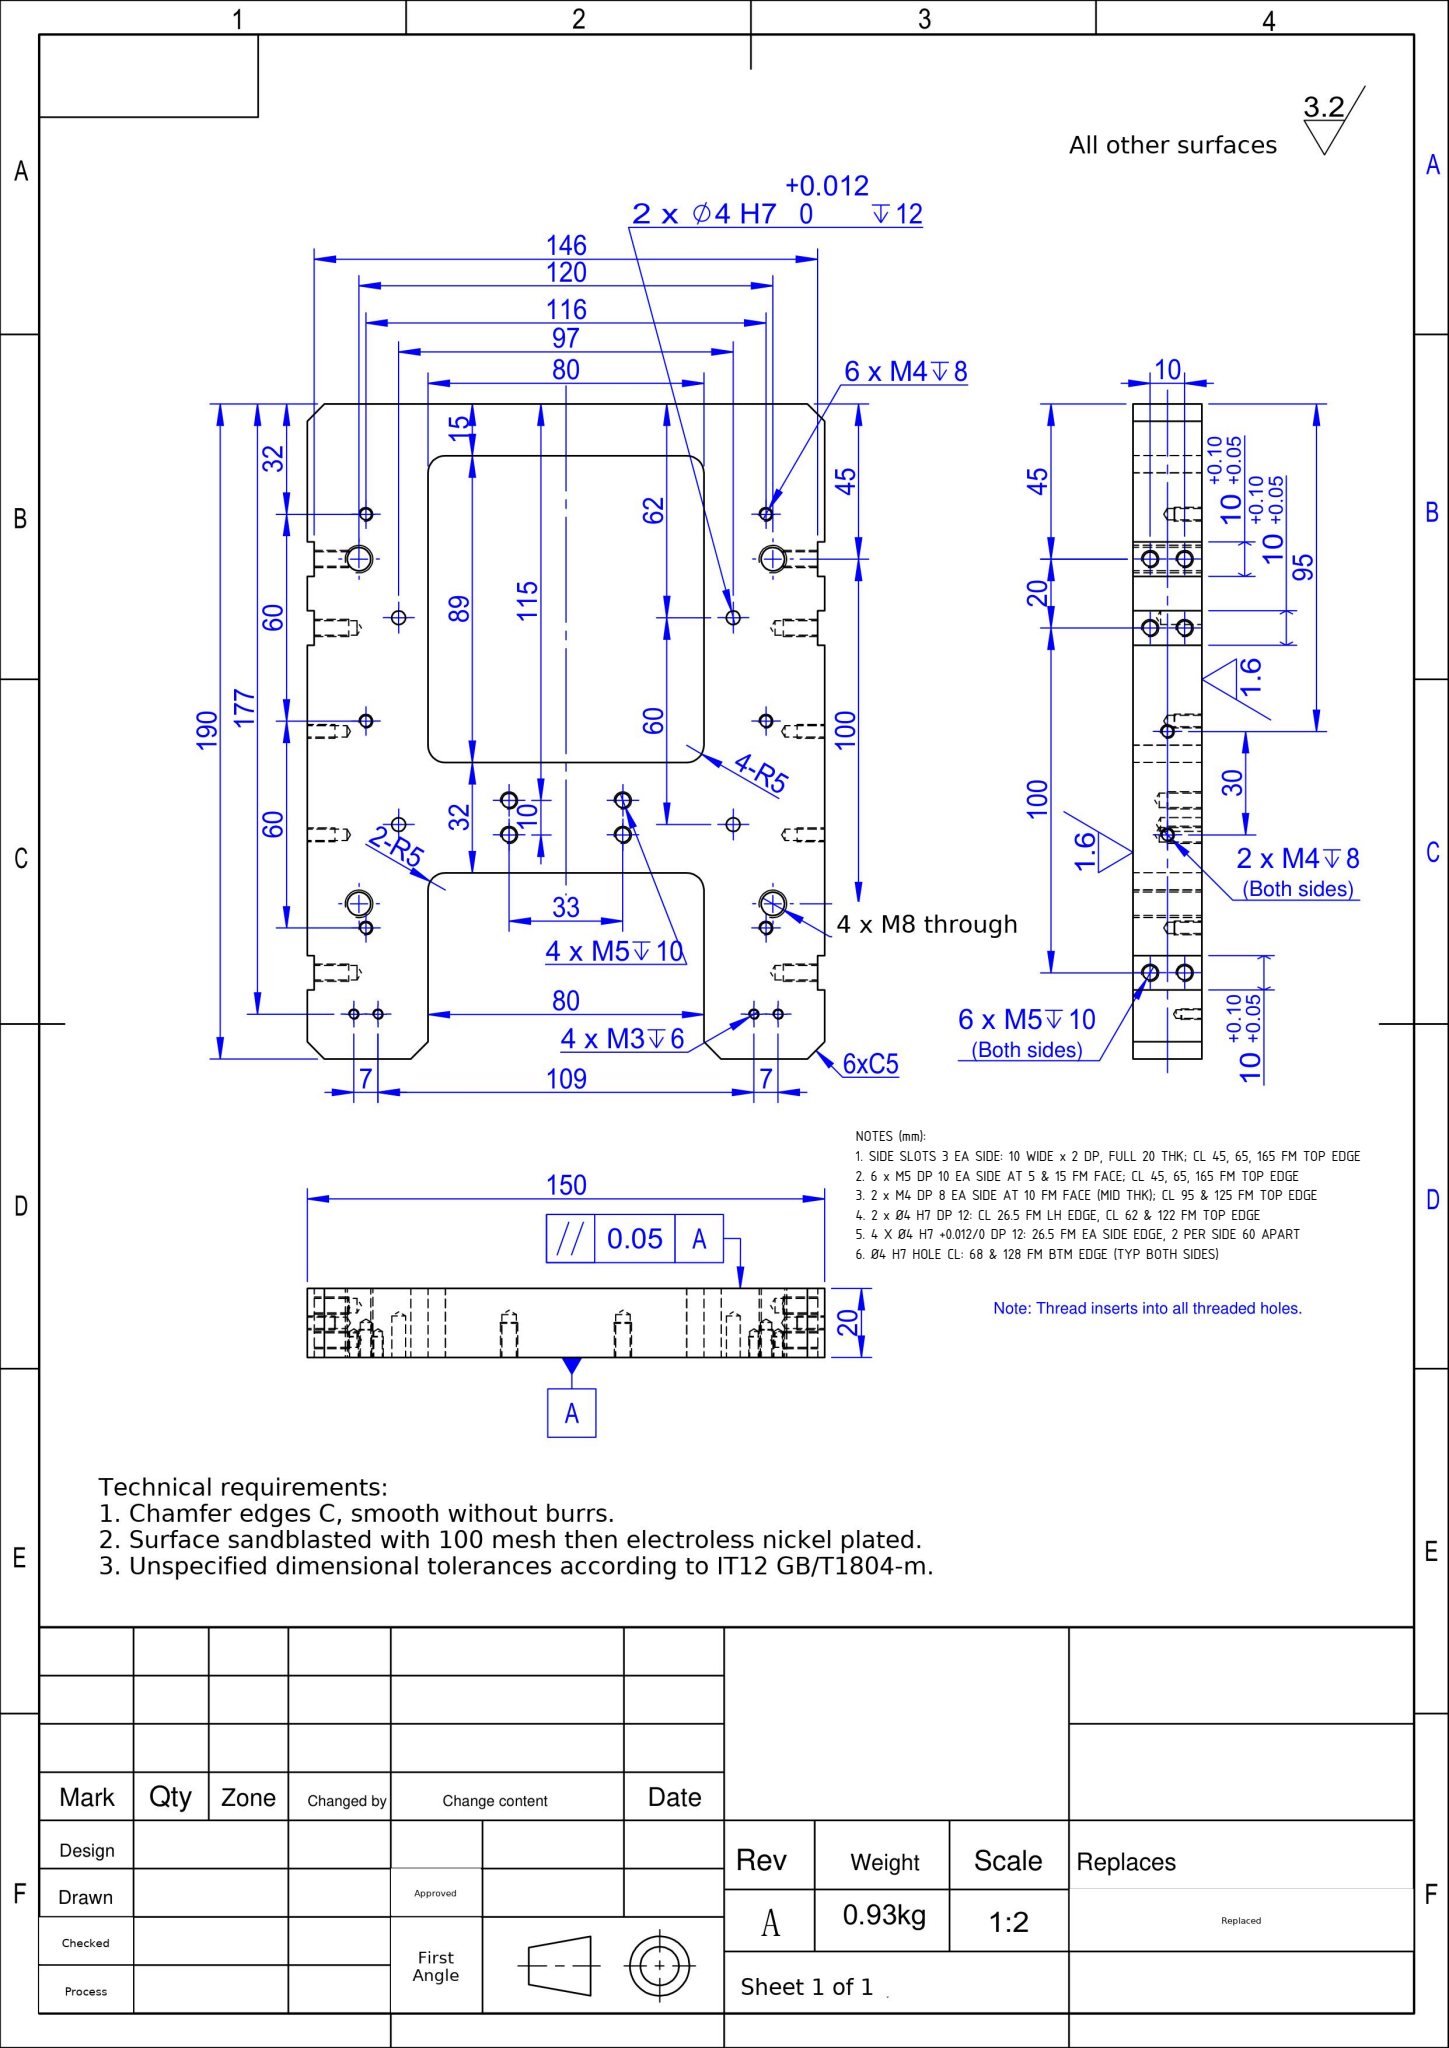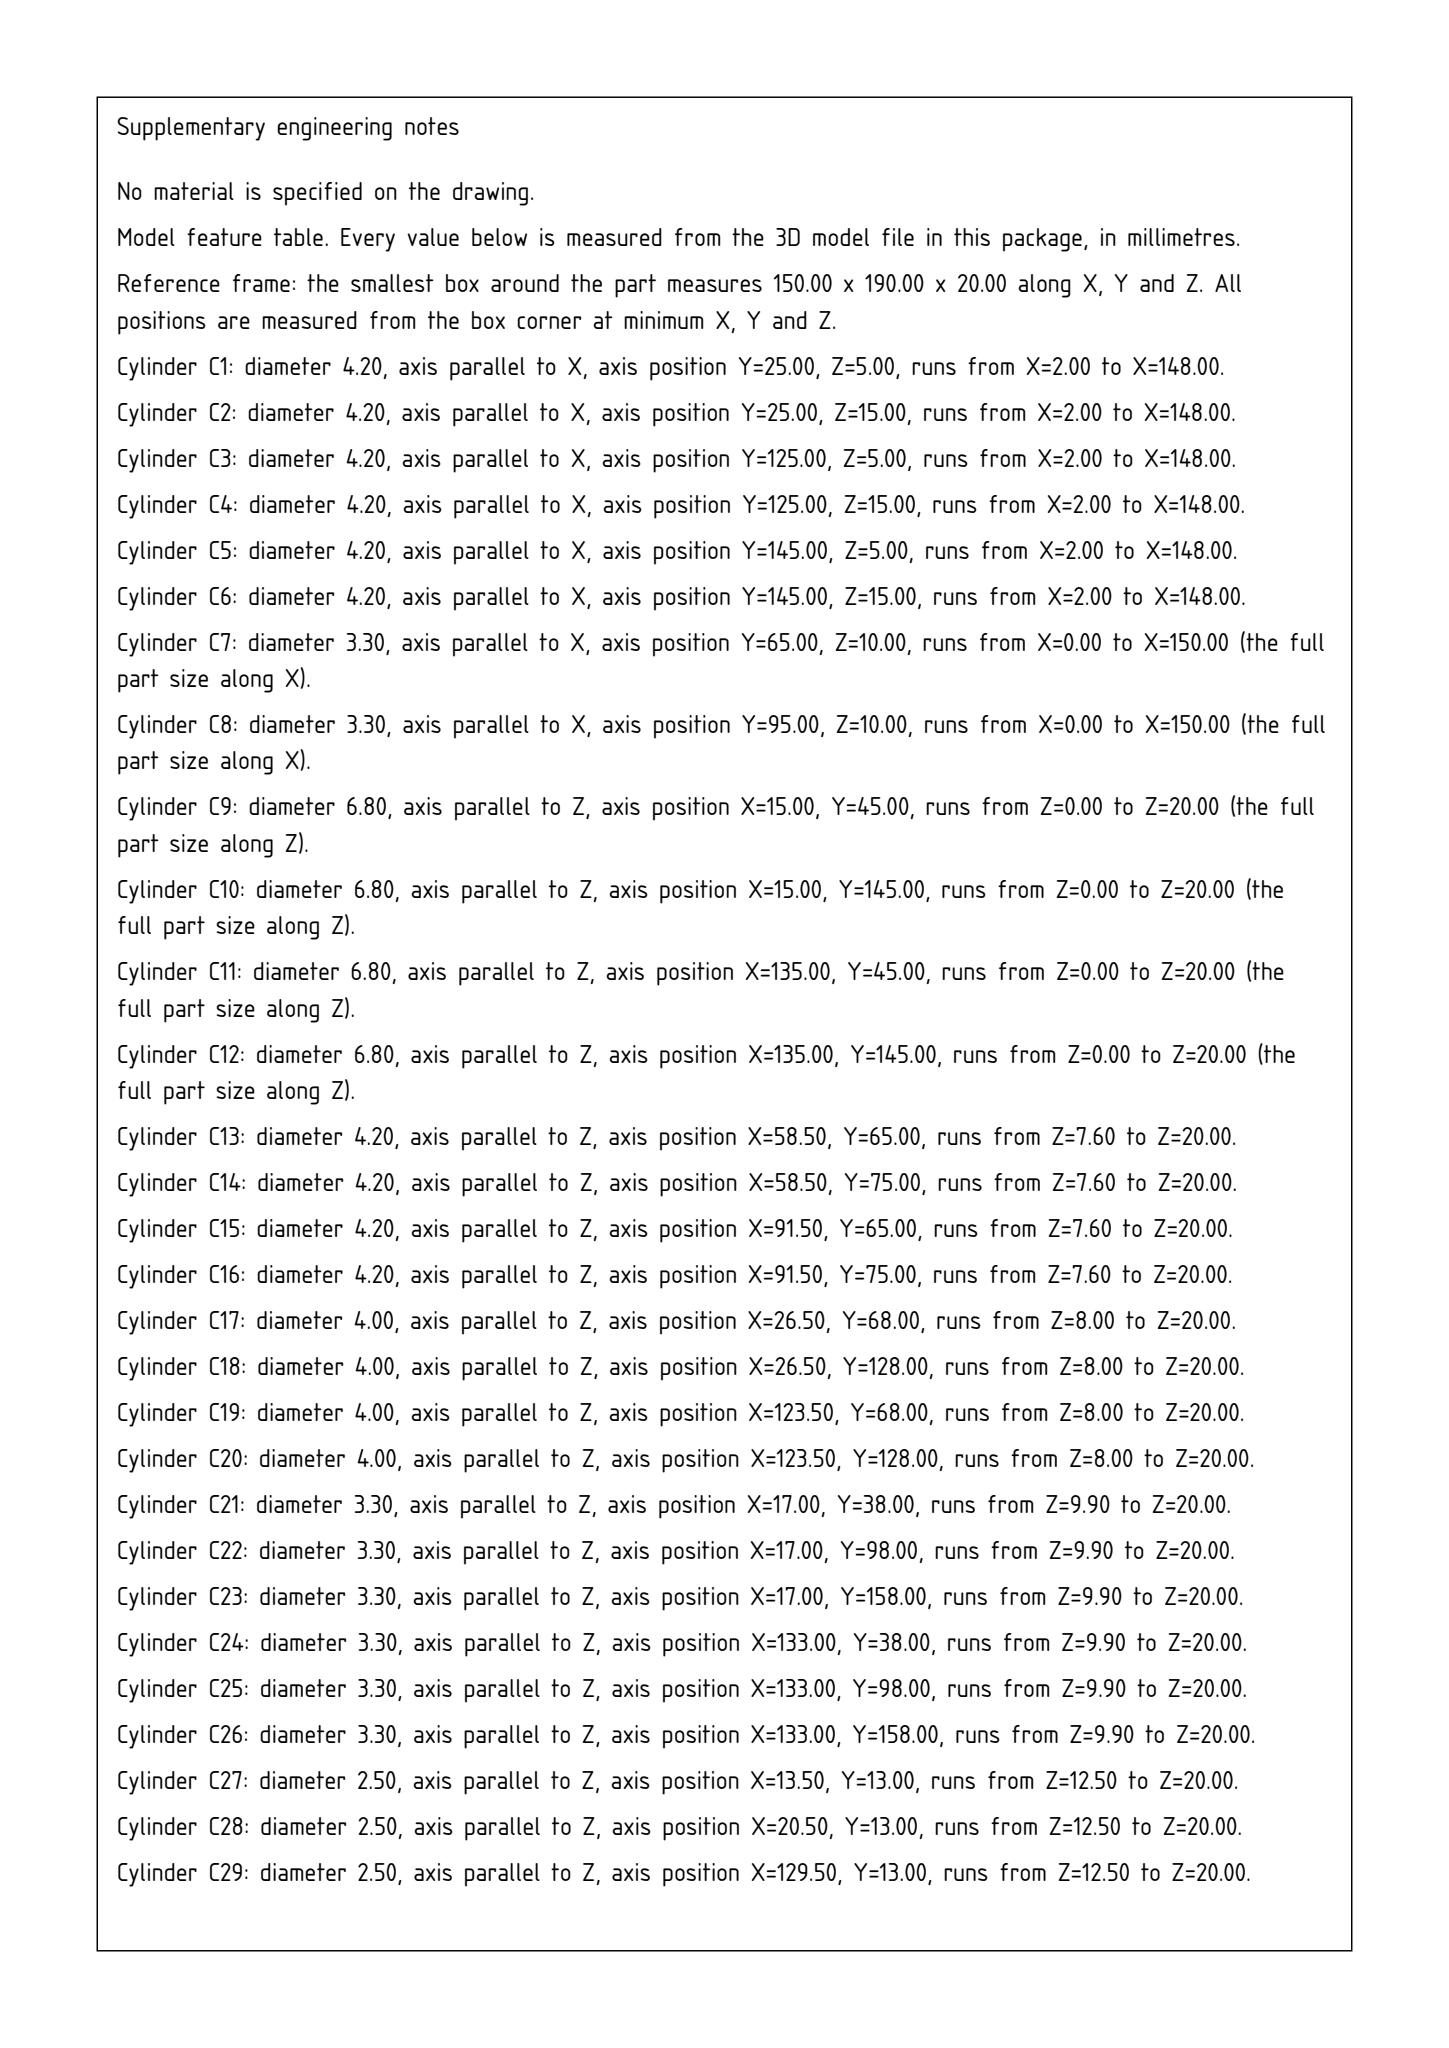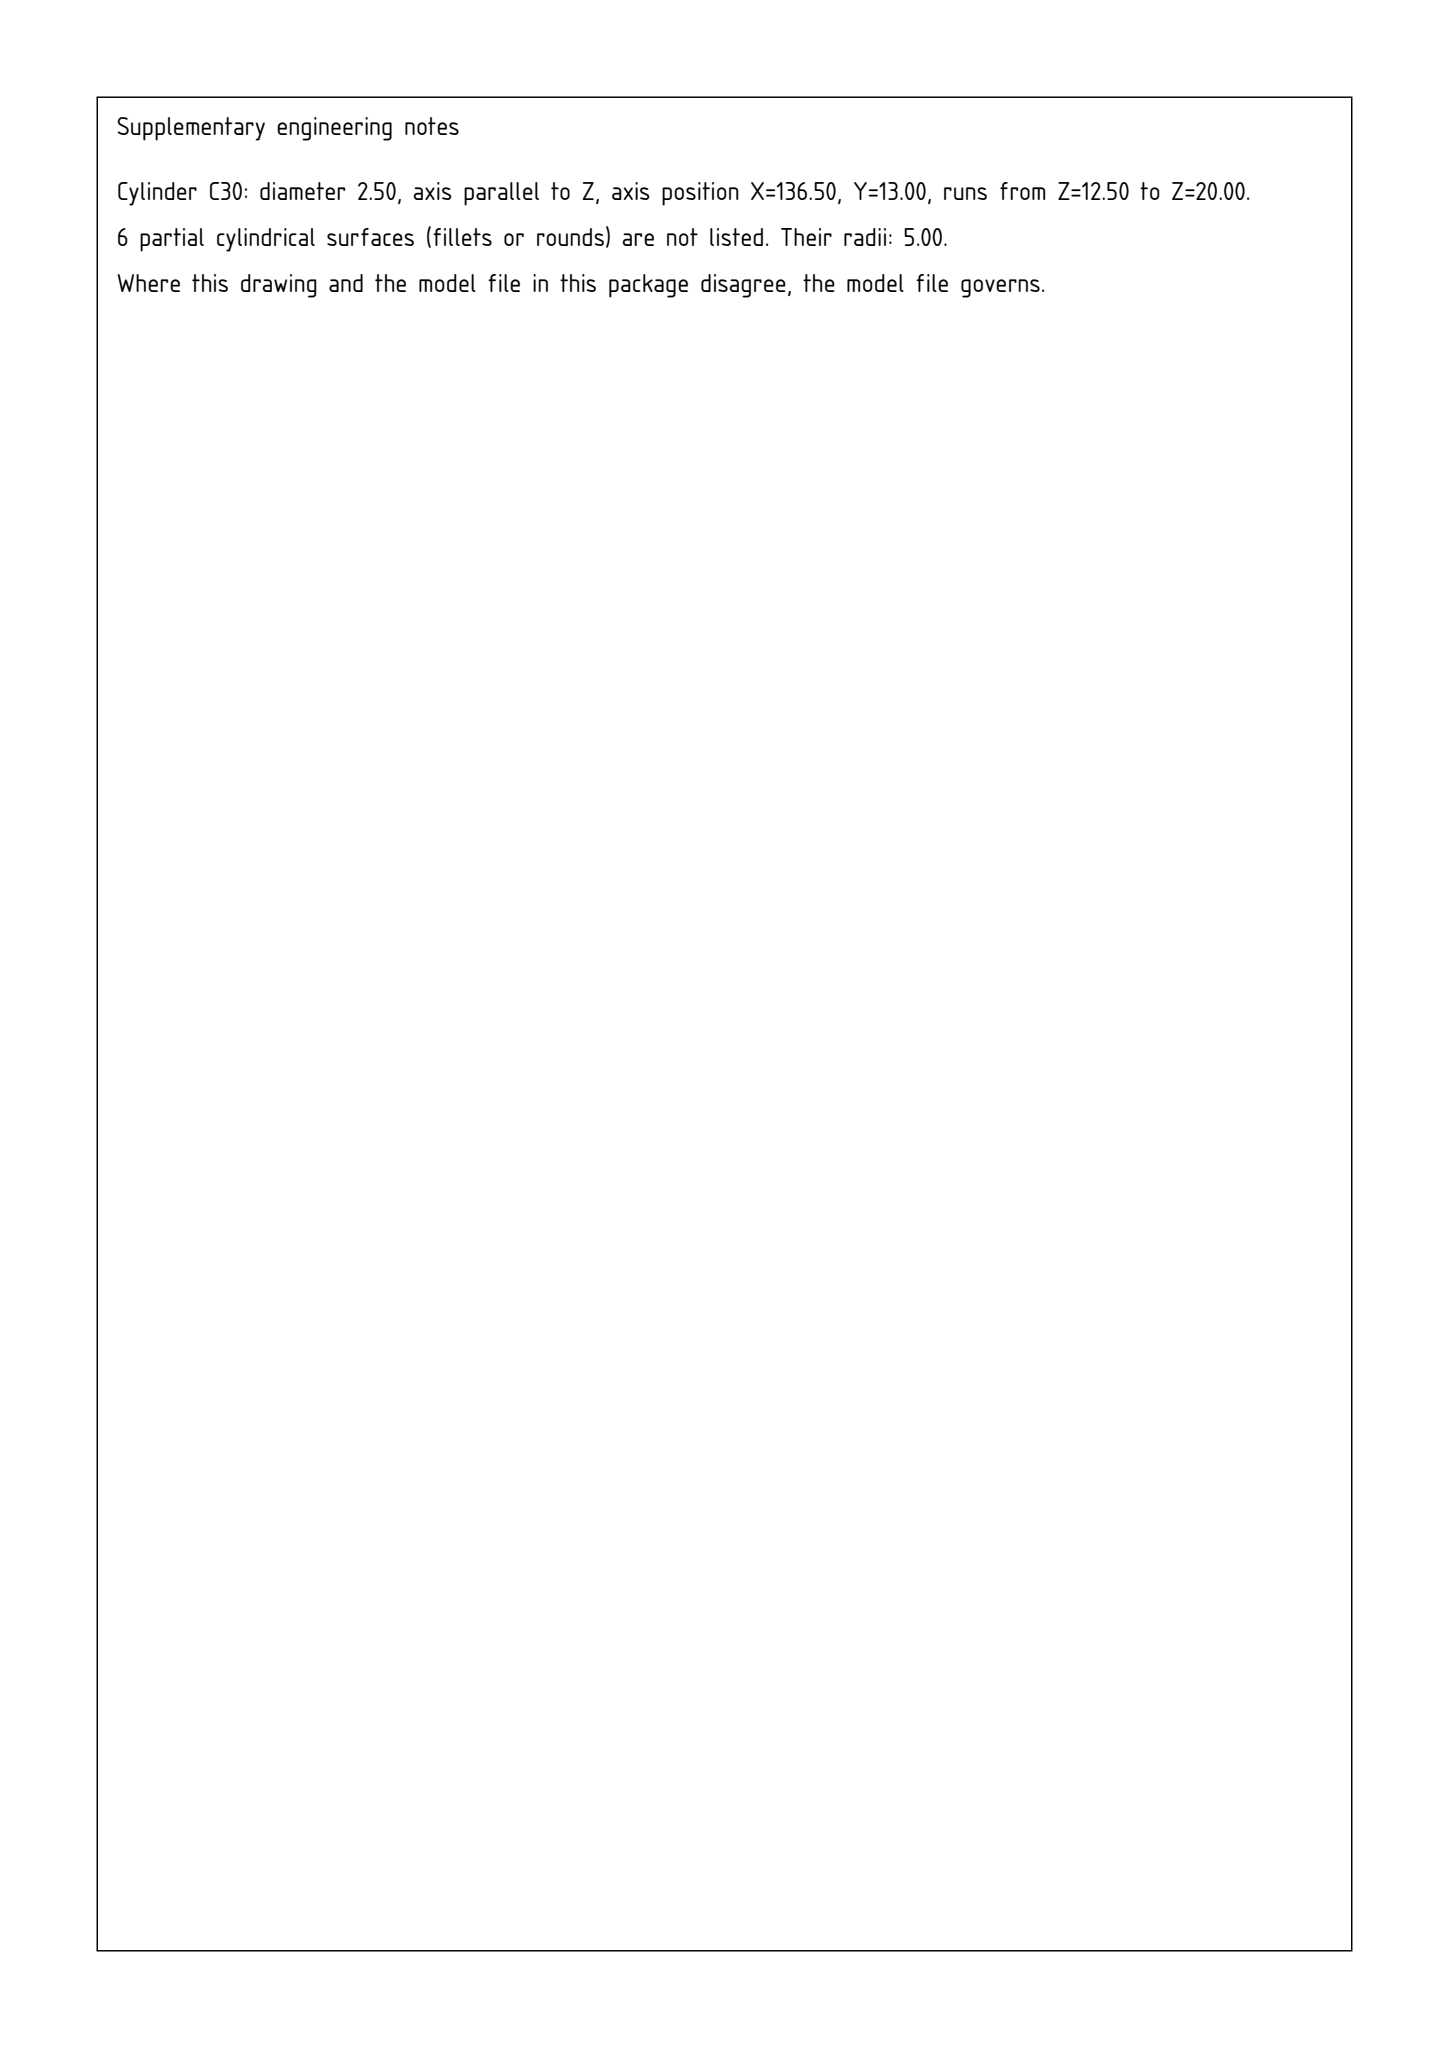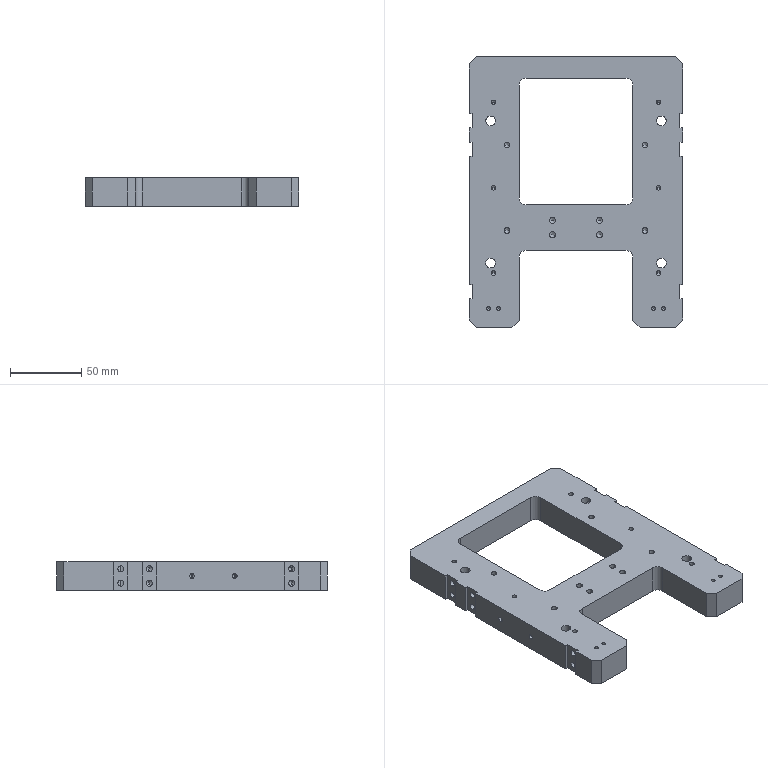Part | SolidWorks | mm | 1 solid | 186 faces | box 150 x 190 x 20 mm | volume 330650 mm3 | cylinder 82 | cone 60 | plane 44 | commonest cylinder face diameters 4.2 x32 3.3 x20 4 x8 6.8 x8 2.5 x8 10 x6
Drawing notes:
SIDE SLOTS 3 EA SIDE: 10 WIDE x 2 DP, FULL 20 THK; CL 45, 65, 165 FM TOP EDGE | from the solid: x-normal planes at 2.0 & 148.0 vs faces x=0/150 -> 2 deep; y pairs 20-30, 120-130, 140-150 -> 10 wide; z 0-20 full thk; slot CL y=145/125/25 -> 190-y = 45/65/165
6 x M5 DP 10 EA SIDE AT 5 & 15 FM FACE; CL 45, 65, 165 FM TOP EDGE | from the solid: Ø4.2 x-axis holes at z=5 and z=15 in 20 thk; at y=145, 125, 25 -> 190-y = 45, 65, 165
2 x M4 DP 8 EA SIDE AT 10 FM FACE (MID THK); CL 95 & 125 FM TOP EDGE | from the solid: Ø3.3 x-axis holes at z=10.0, y=95 and y=65 -> 190-y = 95 and 125
2 x Ø4 H7 DP 12: CL 26.5 FM LH EDGE, CL 62 & 122 FM TOP EDGE | from the solid: dia 4.0 z-holes, x=26.5, y=128 (190-128=62) and y=68 (190-68=122), length 12
4 X Ø4 H7 +0.012/0 DP 12: 26.5 FM EA SIDE EDGE, 2 PER SIDE 60 APART | from the solid: Ø4.0 z-axis holes at (26.5,68),(26.5,128),(123.5,68),(123.5,128), L=12; bbox X=150 so 150-123.5=26.5
Ø4 H7 HOLE CL: 68 & 128 FM BTM EDGE (TYP BOTH SIDES) | from the solid: Ø4.0 holes y=68 and y=128 from bbox Y min; bbox Y=190
build123d program:
from build123d import *

# Parameters (mm, degrees)
SKETCH1_W                         = 150
SKETCH1_H                         = 20
BOSS_EXTRUDE1_DEPTH               = 190
M4_TAPPED_HOLE1_D                 = 3.3
M4_TAPPED_HOLE1_DEPTH             = 10.1
M4_TAPPED_HOLE1_TIP               = 0.9914
M3_TAPPED_HOLE1_D                 = 2.5
M3_TAPPED_HOLE1_DEPTH             = 7.5
M3_TAPPED_HOLE1_TIP               = 0.7511
M5_TAPPED_HOLE1_AT_2_COUNT        = 2
M5_TAPPED_HOLE1_AT_2_PITCH        = 33
CUT_EXTRUDE2_DEPTH                = 206.244
M8_TAPPED_HOLE1_D                 = 6.8
LPATTERN1_COUNT                   = 2
LPATTERN1_PITCH                   = 100
LPATTERN1_COPY_1_D                = 6.8
CHAMFER2_SIZE                     = 5
SKETCH23_W                        = 2
SKETCH23_H                        = 10
CUT_EXTRUDE3_DEPTH                = 206.244
SKETCH24_W                        = 20
SKETCH24_H                        = 10
CUT_EXTRUDE4_DEPTH                = 2
M5_TAPPED_HOLE2_AT_2_COUNT        = 2
M5_TAPPED_HOLE2_AT_2_PITCH        = 10
M5_TAPPED_HOLE2_AT_3_COUNT        = 2
M5_TAPPED_HOLE2_AT_3_PITCH        = 120.416
M5_TAPPED_HOLE2_AT_4_COUNT        = 2
M5_TAPPED_HOLE2_AT_4_PITCH        = 120
M5_TAPPED_HOLE2_AT_5_COUNT        = 2
M5_TAPPED_HOLE2_AT_5_PITCH        = 22.361
M5_TAPPED_HOLE2_AT_6_COUNT        = 2
M5_TAPPED_HOLE2_AT_6_PITCH        = 20
M4_TAPPED_HOLE2_AT_2_COUNT        = 2
M4_TAPPED_HOLE2_AT_2_PITCH        = 30
LPATTERN2_COUNT                   = 2
LPATTERN2_PITCH                   = 10
F_4_0_4_DIAMETER_HOLE1_AT_2_COUNT = 2
F_4_0_4_DIAMETER_HOLE1_AT_2_PITCH = 60


with BuildPart() as part:
    # Sketch1 → Boss-Extrude1 (new body)
    with BuildSketch(Plane(origin=(0, 0, 0), x_dir=(1, 0, 0), z_dir=(0, 1, 0))):
        Rectangle(SKETCH1_W, SKETCH1_H)
    extrude(amount=BOSS_EXTRUDE1_DEPTH)

    # M4 Tapped Hole1
    with Locations(Plane.XY.offset(10)):
        with Locations((-58, 38), (-58, 98), (-58, 158), (58, 158), (58, 98), (58, 38)):
            Hole(M4_TAPPED_HOLE1_D / 2, depth=M4_TAPPED_HOLE1_DEPTH)
            with Locations((0, 0, -(M4_TAPPED_HOLE1_DEPTH + M4_TAPPED_HOLE1_TIP / 2))):  # 118° drill point
                Cone(0, M4_TAPPED_HOLE1_D / 2, M4_TAPPED_HOLE1_TIP, mode=Mode.SUBTRACT)

    # M3 Tapped Hole1
    with Locations(Plane.XY.offset(10)):
        with Locations((54.5, 13), (61.5, 13), (-61.5, 13), (-54.5, 13)):
            Hole(M3_TAPPED_HOLE1_D / 2, depth=M3_TAPPED_HOLE1_DEPTH)
            with Locations((0, 0, -(M3_TAPPED_HOLE1_DEPTH + M3_TAPPED_HOLE1_TIP / 2))):  # 118° drill point
                Cone(0, M3_TAPPED_HOLE1_D / 2, M3_TAPPED_HOLE1_TIP, mode=Mode.SUBTRACT)

    # Sketch9 → M5 Tapped Hole1 (revolve, cut)
    with BuildSketch(Plane(origin=(-16.5, 65, 10), x_dir=(0, -1, 0), z_dir=(1, 0, 0))):
        Polygon((0, 0), (0, 13.662), (2.1, 12.4), (2.1, 0), align=None)
    m5_tapped_hole1 = revolve(axis=Axis((-16.5, 65, 16.35), (0, 0, -1)), mode=Mode.SUBTRACT)

    # M5 Tapped Hole1 at 2: M5 Tapped Hole1 ×2
    with Locations(*[(i * M5_TAPPED_HOLE1_AT_2_PITCH, 0, 0) for i in range(1, M5_TAPPED_HOLE1_AT_2_COUNT)]):
        add(m5_tapped_hole1, mode=Mode.SUBTRACT)

    # Sketch11 → Cut-Extrude2 (cut, through all)
    with BuildSketch(Plane.XY.offset(10)):
        with BuildLine():
            Line((-35, 175), (35, 175))
            ThreePointArc((35, 175), (38.536, 173.536), (40, 170))
            Line((40, 170), (40, 91))
            ThreePointArc((40, 91), (38.536, 87.464), (35, 86))
            Line((35, 86), (-35, 86))
            ThreePointArc((-35, 86), (-38.536, 87.464), (-40, 91))
            Line((-40, 91), (-40, 170))
            ThreePointArc((-40, 170), (-38.536, 173.536), (-35, 175))
        make_face()
        with BuildLine():
            Line((-35, 54), (35, 54))
            ThreePointArc((35, 54), (38.536, 52.536), (40, 49))
            Line((40, 49), (40, 0))
            Line((40, 0), (-40, 0))
            Line((-40, 0), (-40, 49))
            ThreePointArc((-40, 49), (-38.536, 52.536), (-35, 54))
        make_face()
    extrude(amount=-CUT_EXTRUDE2_DEPTH, mode=Mode.SUBTRACT)

    # M8 Tapped Hole1 (through all)
    with Locations(Plane(origin=(116.284, -1.864, 10), x_dir=(-1, 0, 0), z_dir=(0, 0, 1))):
        with Locations((176.284, -146.864)):
            m8_tapped_hole1 = Hole(M8_TAPPED_HOLE1_D / 2)

    # Mirror2: M8 Tapped Hole1 across plane
    add(m8_tapped_hole1.mirror(Plane(origin=(0, 0, 0), x_dir=(0, 0, 1), z_dir=(1, 0, 0))), mode=Mode.SUBTRACT)

    # LPattern1: M8 Tapped Hole1 ×2
    with Locations(*[(0, -i * LPATTERN1_PITCH, 0) for i in range(1, LPATTERN1_COUNT)]):
        add(m8_tapped_hole1, mode=Mode.SUBTRACT)

    # LPattern1 copy 1 (through all)
    with Locations(Plane(origin=(-116.284, -101.864, 10), x_dir=(1, 0, 0), z_dir=(0, 0, 1))):
        with Locations((176.284, 146.864)):
            Hole(LPATTERN1_COPY_1_D / 2)

    # Chamfer2
    chamfer2_edges = [part.edges().sort_by_distance(p)[0] for p in [
        (75, 190, 0),
        (-75, 190, 0),
        (75, 0, 0),
        (-75, 0, 0),
        (40, 0, 0),
        (-40, 0, 0),
    ]]
    chamfer(chamfer2_edges, length=CHAMFER2_SIZE)

    # Sketch23 → Cut-Extrude3 (cut, through all)
    with BuildSketch(Plane.XY.offset(10)):
        with Locations((-74, 25)):
            Rectangle(SKETCH23_W, SKETCH23_H)
    cut_extrude3 = extrude(amount=-CUT_EXTRUDE3_DEPTH, mode=Mode.SUBTRACT)

    # Sketch24 → Cut-Extrude4 (cut)
    with BuildSketch(Plane.ZY.offset(75)):
        with Locations((0, 145)):
            Rectangle(SKETCH24_W, SKETCH24_H)
        with Locations((0, 125)):
            Rectangle(SKETCH24_W, SKETCH24_H)
    cut_extrude4 = extrude(amount=-CUT_EXTRUDE4_DEPTH, mode=Mode.SUBTRACT)

    # Sketch25 → M5 Tapped Hole2 (revolve, cut)
    with BuildSketch(Plane(origin=(-73, 145, 5), x_dir=(0, 0, 1), z_dir=(0, 1, 0))):
        Polygon((0, 0), (0, 13.662), (2.1, 12.4), (2.1, 0), align=None)
    m5_tapped_hole2 = revolve(axis=Axis((-79.35, 145, 5), (1, 0, 0)), mode=Mode.SUBTRACT)

    # M5 Tapped Hole2 at 2: M5 Tapped Hole2 ×2
    with Locations(*[(0, 0, -i * M5_TAPPED_HOLE2_AT_2_PITCH) for i in range(1, M5_TAPPED_HOLE2_AT_2_COUNT)]):
        add(m5_tapped_hole2, mode=Mode.SUBTRACT)

    # M5 Tapped Hole2 at 3: M5 Tapped Hole2 ×2
    with Locations(*[Vector(0, -0.9965, -0.08305) * (i * M5_TAPPED_HOLE2_AT_3_PITCH) for i in range(1, M5_TAPPED_HOLE2_AT_3_COUNT)]):
        add(m5_tapped_hole2, mode=Mode.SUBTRACT)

    # M5 Tapped Hole2 at 4: M5 Tapped Hole2 ×2
    with Locations(*[(0, -i * M5_TAPPED_HOLE2_AT_4_PITCH, 0) for i in range(1, M5_TAPPED_HOLE2_AT_4_COUNT)]):
        add(m5_tapped_hole2, mode=Mode.SUBTRACT)

    # M5 Tapped Hole2 at 5: M5 Tapped Hole2 ×2
    with Locations(*[Vector(0, -0.8944, -0.4472) * (i * M5_TAPPED_HOLE2_AT_5_PITCH) for i in range(1, M5_TAPPED_HOLE2_AT_5_COUNT)]):
        add(m5_tapped_hole2, mode=Mode.SUBTRACT)

    # M5 Tapped Hole2 at 6: M5 Tapped Hole2 ×2
    with Locations(*[(0, -i * M5_TAPPED_HOLE2_AT_6_PITCH, 0) for i in range(1, M5_TAPPED_HOLE2_AT_6_COUNT)]):
        add(m5_tapped_hole2, mode=Mode.SUBTRACT)

    # Mirror3: Cut-Extrude3, Cut-Extrude4, M5 Tapped Hole2 across plane
    add(cut_extrude3.mirror(Plane(origin=(0, 0, 0), x_dir=(0, 0, 1), z_dir=(1, 0, 0))), mode=Mode.SUBTRACT)
    add(cut_extrude4.mirror(Plane(origin=(0, 0, 0), x_dir=(0, 0, 1), z_dir=(1, 0, 0))), mode=Mode.SUBTRACT)
    add(m5_tapped_hole2.mirror(Plane(origin=(0, 0, 0), x_dir=(0, 0, 1), z_dir=(1, 0, 0))), mode=Mode.SUBTRACT)

    # Mirror3 copy 1 sketch → Mirror3 copy 1 (revolve, cut)
    with BuildSketch(Plane(origin=(73, 145, -5), x_dir=(0, 0, 1), z_dir=(0, 1, 0))):
        Polygon((0, 0), (0, -13.662), (2.1, -12.4), (2.1, 0), align=None)
    revolve(axis=Axis((79.35, 145, -5), (1, 0, 0)), mode=Mode.SUBTRACT)

    # Mirror3 copy 2 sketch → Mirror3 copy 2 (revolve, cut)
    with BuildSketch(Plane(origin=(73, 25, -5), x_dir=(0, 0, 1), z_dir=(0, 1, 0))):
        Polygon((0, 0), (0, -13.662), (2.1, -12.4), (2.1, 0), align=None)
    revolve(axis=Axis((79.35, 25, -5), (1, 0, 0)), mode=Mode.SUBTRACT)

    # Mirror3 copy 3 sketch → Mirror3 copy 3 (revolve, cut)
    with BuildSketch(Plane(origin=(73, 25, 5), x_dir=(0, 0, 1), z_dir=(0, 1, 0))):
        Polygon((0, 0), (0, -13.662), (2.1, -12.4), (2.1, 0), align=None)
    revolve(axis=Axis((79.35, 25, 5), (1, 0, 0)), mode=Mode.SUBTRACT)

    # Mirror3 copy 4 sketch → Mirror3 copy 4 (revolve, cut)
    with BuildSketch(Plane(origin=(73, 125, -5), x_dir=(0, 0, 1), z_dir=(0, 1, 0))):
        Polygon((0, 0), (0, -13.662), (2.1, -12.4), (2.1, 0), align=None)
    revolve(axis=Axis((79.35, 125, -5), (1, 0, 0)), mode=Mode.SUBTRACT)

    # Mirror3 copy 5 sketch → Mirror3 copy 5 (revolve, cut)
    with BuildSketch(Plane(origin=(73, 125, 5), x_dir=(0, 0, 1), z_dir=(0, 1, 0))):
        Polygon((0, 0), (0, -13.662), (2.1, -12.4), (2.1, 0), align=None)
    revolve(axis=Axis((79.35, 125, 5), (1, 0, 0)), mode=Mode.SUBTRACT)

    # Sketch29 → M4 Tapped Hole2 (revolve, cut)
    with BuildSketch(Plane(origin=(75, 65, 0), x_dir=(0, 0, -1), z_dir=(0, 1, 0))):
        Polygon((0, 0), (0, 12.491), (1.65, 11.5), (1.65, 0), align=None)
    m4_tapped_hole2 = revolve(axis=Axis((81.35, 65, 0), (-1, 0, 0)), mode=Mode.SUBTRACT)

    # M4 Tapped Hole2 at 2: M4 Tapped Hole2 ×2
    with Locations(*[(0, i * M4_TAPPED_HOLE2_AT_2_PITCH, 0) for i in range(1, M4_TAPPED_HOLE2_AT_2_COUNT)]):
        add(m4_tapped_hole2, mode=Mode.SUBTRACT)

    # Mirror4: M4 Tapped Hole2 across plane
    add(m4_tapped_hole2.mirror(Plane(origin=(0, 0, 0), x_dir=(0, 0, 1), z_dir=(1, 0, 0))), mode=Mode.SUBTRACT)

    # Mirror4 copy 1 sketch → Mirror4 copy 1 (revolve, cut)
    with BuildSketch(Plane(origin=(-75, 95, 0), x_dir=(0, 0, -1), z_dir=(0, 1, 0))):
        Polygon((0, 0), (0, -12.491), (1.65, -11.5), (1.65, 0), align=None)
    revolve(axis=Axis((-81.35, 95, 0), (-1, 0, 0)), mode=Mode.SUBTRACT)

    # LPattern2: M5 Tapped Hole1 ×2
    with Locations(*[(0, i * LPATTERN2_PITCH, 0) for i in range(1, LPATTERN2_COUNT)]):
        add(m5_tapped_hole1, mode=Mode.SUBTRACT)

    # LPattern2 copy 1 sketch → LPattern2 copy 1 (revolve, cut)
    with BuildSketch(Plane(origin=(16.5, 75, 10), x_dir=(0, -1, 0), z_dir=(1, 0, 0))):
        Polygon((0, 0), (0, 13.662), (2.1, 12.4), (2.1, 0), align=None)
    revolve(axis=Axis((16.5, 75, 16.35), (0, 0, -1)), mode=Mode.SUBTRACT)

    # Sketch31 → 4.0 _4_ Diameter Hole1 (revolve, cut)
    with BuildSketch(Plane(origin=(48.5, 128, 10), x_dir=(0, -1, 0), z_dir=(1, 0, 0))):
        Polygon((0, 0), (0, 13.202), (2, 12), (2, 0), align=None)
    f_4_0_4_diameter_hole1 = revolve(axis=Axis((48.5, 128, 16.35), (0, 0, -1)), mode=Mode.SUBTRACT)

    # 4.0 _4_ Diameter Hole1 at 2: 4.0 _4_ Diameter Hole1 ×2
    with Locations(*[(0, -i * F_4_0_4_DIAMETER_HOLE1_AT_2_PITCH, 0) for i in range(1, F_4_0_4_DIAMETER_HOLE1_AT_2_COUNT)]):
        add(f_4_0_4_diameter_hole1, mode=Mode.SUBTRACT)

    # Mirror5: 4.0 _4_ Diameter Hole1 across plane
    add(f_4_0_4_diameter_hole1.mirror(Plane(origin=(0, 0, 0), x_dir=(0, 0, 1), z_dir=(1, 0, 0))), mode=Mode.SUBTRACT)

    # Mirror5 copy 1 sketch → Mirror5 copy 1 (revolve, cut)
    with BuildSketch(Plane(origin=(-48.5, 68, 10), x_dir=(0, -1, 0), z_dir=(-1, 0, 0))):
        Polygon((0, 0), (0, -13.202), (2, -12), (2, 0), align=None)
    revolve(axis=Axis((-48.5, 68, 16.35), (0, 0, 1)), mode=Mode.SUBTRACT)


solid = part.part